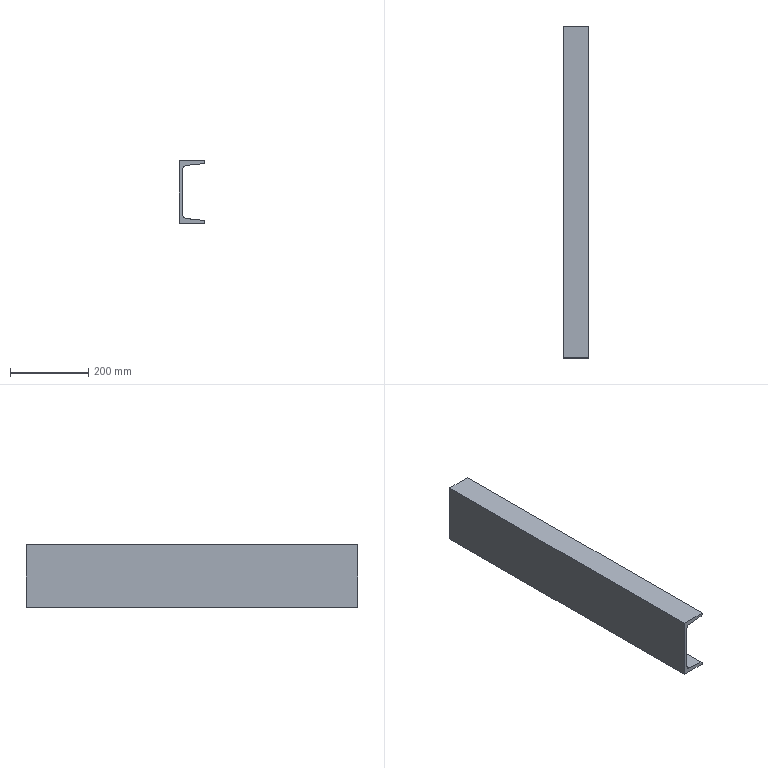Component | SolidWorks | NitrogenSupportChannelSteel65016a-2-331MachineTool-1 | 1 solid | 16 faces | box 65 x 850 x 160 mm | volume 2137912 mm3 | plane 10 | cylinder 6 | commonest cylinder face diameters 5 x2 20 x2 10 x2
build123d program:
from build123d import *

# Parameters (mm, degrees)
BOSS_EXTRUDE1_DEPTH    = 850
M6_TAPPED_HOLE1_REACH  = 866.871
M6_TAPPED_HOLE1_BORE_R = 2.5


with BuildPart() as part:
    # Sketch1 → Boss-Extrude1 (new body)
    with BuildSketch(Plane(origin=(0, 0, 0), x_dir=(-1, 0, 0), z_dir=(0, 0, -1))):
        with BuildLine():
            Line((-8.5, 138.125), (-8.5, 21.875))
            ThreePointArc((-8.5, 21.875), (-11.085, 15.165), (-17.505, 11.925))
            Line((-17.505, 11.925), (-60.498, 7.625))
            ThreePointArc((-60.498, 7.625), (-63.707, 6.005), (-65, 2.65))
            Line((-65, 2.65), (-65, 0))
            Line((-65, 0), (0, 0))
            Line((0, 0), (0, 160))
            Line((0, 160), (-65, 160))
            Line((-65, 160), (-65, 157.35))
            ThreePointArc((-65, 157.35), (-63.707, 153.995), (-60.498, 152.375))
            Line((-60.498, 152.375), (-17.505, 148.075))
            ThreePointArc((-17.505, 148.075), (-11.085, 144.835), (-8.5, 138.125))
        make_face()
    extrude(amount=-BOSS_EXTRUDE1_DEPTH)

    # M6 Tapped Hole1 bore → M6 Tapped Hole1 (cut, up to next)
    with BuildSketch(Plane(origin=(1.354, 13.54, 0), x_dir=(0.995, -0.0995, 0), z_dir=(0.0995, 0.995, 0)), mode=Mode.PRIVATE) as m6_tapped_hole1_sk1:
        with Locations((39.487, -548.988)):
            Circle(M6_TAPPED_HOLE1_BORE_R)
    m6_tapped_hole1_tool1 = extrude(m6_tapped_hole1_sk1.sketch, amount=-M6_TAPPED_HOLE1_REACH, mode=Mode.PRIVATE) & part.part
    add(m6_tapped_hole1_tool1.solids().sort_by_distance((40.645, 9.61, 548.988))[0], mode=Mode.SUBTRACT)


solid = part.part

# Placed as in the assembly
solid = solid.moved(Location((-286.681, 723.438, 590), (90, 0, 0)))
STEP:
#1=CARTESIAN_POINT('',(-9.823,6.868,23.228));
#2=VERTEX_POINT('',#1);
#3=CARTESIAN_POINT('',(-9.625,6.868,23.228));
#4=VERTEX_POINT('',#3);
#5=CARTESIAN_POINT('',(-9.823,6.868,23.228));
#6=CARTESIAN_POINT('',(-9.823,7.065,23.228));
#7=CARTESIAN_POINT('',(-9.625,7.065,23.228));
#8=CARTESIAN_POINT('',(-9.625,6.868,23.228));
#9=(BOUNDED_CURVE()B_SPLINE_CURVE(3,(#5,#6,#7,#8),.UNSPECIFIED.,.F.,.T.)B_SPLINE_CURVE_WITH_KNOTS((4,4),(3.142,6.283),.UNSPECIFIED.)CURVE()GEOMETRIC_REPRESENTATION_ITEM()RATIONAL_B_SPLINE_CURVE((1.,0.3333,0.3333,1.))REPRESENTATION_ITEM(''));
#10=EDGE_CURVE('',#2,#4,#9,.T.);
#11=ORIENTED_EDGE('',*,*,#10,.T.);
#12=CARTESIAN_POINT('',(-9.589,6.868,23.597));
#13=VERTEX_POINT('',#12);
#14=CARTESIAN_POINT('',(-9.589,6.868,23.597));
#15=DIRECTION('',(0.0995,-0.,0.995));
#16=VECTOR('',#15,39.37);
#17=LINE('',#14,#16);
#18=EDGE_CURVE('',#4,#13,#17,.T.);
#19=ORIENTED_EDGE('',*,*,#18,.T.);
#20=CARTESIAN_POINT('',(-9.784,6.868,23.617));
#21=VERTEX_POINT('',#20);
#22=CARTESIAN_POINT('',(-9.686,6.868,23.607));
#23=DIRECTION('',(0.0995,-0.,0.995));
#24=DIRECTION('',(-0.995,0.,0.0995));
#25=AXIS2_PLACEMENT_3D('',#22,#23,#24);
#26=CIRCLE('',#25,0.09843);
#27=EDGE_CURVE('',#13,#21,#26,.T.);
#28=ORIENTED_EDGE('',*,*,#27,.T.);
#29=CARTESIAN_POINT('',(-9.784,6.868,23.617));
#30=DIRECTION('',(0.0995,-0.,0.995));
#31=VECTOR('',#30,39.37);
#32=LINE('',#29,#31);
#33=EDGE_CURVE('',#2,#21,#32,.T.);
#34=ORIENTED_EDGE('',*,*,#33,.F.);
#35=EDGE_LOOP('',(#11,#19,#28,#34));
#36=FACE_OUTER_BOUND('',#35,.T.);
#37=CARTESIAN_POINT('',(-9.686,6.868,23.607));
#38=DIRECTION('',(0.0995,-0.,0.995));
#39=DIRECTION('',(-0.995,0.,0.0995));
#40=AXIS2_PLACEMENT_3D('',#37,#38,#39);
#41=CYLINDRICAL_SURFACE('',#40,0.09843);
#42=ADVANCED_FACE('',(#36),#41,.F.);
#43=CARTESIAN_POINT('',(-10.597,28.482,29.058));
#44=VERTEX_POINT('',#43);
#45=CARTESIAN_POINT('',(-10.952,28.482,28.666));
#46=VERTEX_POINT('',#45);
#47=CARTESIAN_POINT('',(-10.558,28.482,28.666));
#48=DIRECTION('',(-0.,-1.,-0.));
#49=DIRECTION('',(1.,0.,0.));
#50=AXIS2_PLACEMENT_3D('',#47,#48,#49);
#51=CIRCLE('',#50,0.3937);
#52=EDGE_CURVE('',#44,#46,#51,.T.);
#53=ORIENTED_EDGE('',*,*,#52,.F.);
#54=CARTESIAN_POINT('',(-10.597,-4.983,29.058));
#55=VERTEX_POINT('',#54);
#56=CARTESIAN_POINT('',(-10.597,-4.983,29.058));
#57=DIRECTION('',(0.,1.,0.));
#58=VECTOR('',#57,39.37);
#59=LINE('',#56,#58);
#60=EDGE_CURVE('',#55,#44,#59,.T.);
#61=ORIENTED_EDGE('',*,*,#60,.F.);
#62=CARTESIAN_POINT('',(-10.952,-4.983,28.666));
#63=VERTEX_POINT('',#62);
#64=CARTESIAN_POINT('',(-10.558,-4.983,28.666));
#65=DIRECTION('',(-0.,-1.,-0.));
#66=DIRECTION('',(1.,0.,0.));
#67=AXIS2_PLACEMENT_3D('',#64,#65,#66);
#68=CIRCLE('',#67,0.3937);
#69=EDGE_CURVE('',#55,#63,#68,.T.);
#70=ORIENTED_EDGE('',*,*,#69,.T.);
#71=CARTESIAN_POINT('',(-10.952,-4.983,28.666));
#72=DIRECTION('',(0.,1.,0.));
#73=VECTOR('',#72,39.37);
#74=LINE('',#71,#73);
#75=EDGE_CURVE('',#63,#46,#74,.T.);
#76=ORIENTED_EDGE('',*,*,#75,.T.);
#77=EDGE_LOOP('',(#53,#61,#70,#76));
#78=FACE_OUTER_BOUND('',#77,.T.);
#79=CARTESIAN_POINT('',(-10.558,-4.983,28.666));
#80=DIRECTION('',(0.,1.,0.));
#81=DIRECTION('',(-1.,0.,0.));
#82=AXIS2_PLACEMENT_3D('',#79,#80,#81);
#83=CYLINDRICAL_SURFACE('',#82,0.3937);
#84=ADVANCED_FACE('',(#78),#83,.F.);
#85=CARTESIAN_POINT('',(-8.905,28.482,29.227));
#86=VERTEX_POINT('',#85);
#87=CARTESIAN_POINT('',(-8.905,28.482,29.227));
#88=DIRECTION('',(-0.995,0.,-0.0995));
#89=VECTOR('',#88,39.37);
#90=LINE('',#87,#89);
#91=EDGE_CURVE('',#86,#44,#90,.T.);
#92=ORIENTED_EDGE('',*,*,#91,.F.);
#93=CARTESIAN_POINT('',(-8.905,-4.983,29.227));
#94=VERTEX_POINT('',#93);
#95=CARTESIAN_POINT('',(-8.905,-4.983,29.227));
#96=DIRECTION('',(0.,1.,0.));
#97=VECTOR('',#96,39.37);
#98=LINE('',#95,#97);
#99=EDGE_CURVE('',#94,#86,#98,.T.);
#100=ORIENTED_EDGE('',*,*,#99,.F.);
#101=CARTESIAN_POINT('',(-8.905,-4.983,29.227));
#102=DIRECTION('',(-0.995,0.,-0.0995));
#103=VECTOR('',#102,39.37);
#104=LINE('',#101,#103);
#105=EDGE_CURVE('',#94,#55,#104,.T.);
#106=ORIENTED_EDGE('',*,*,#105,.T.);
#107=ORIENTED_EDGE('',*,*,#60,.T.);
#108=EDGE_LOOP('',(#92,#100,#106,#107));
#109=FACE_OUTER_BOUND('',#108,.T.);
#110=CARTESIAN_POINT('',(-8.905,-4.983,29.227));
#111=DIRECTION('',(0.0995,0.,-0.995));
#112=DIRECTION('',(0.995,-0.,0.0995));
#113=AXIS2_PLACEMENT_3D('',#110,#111,#112);
#114=PLANE('',#113);
#115=ADVANCED_FACE('',(#109),#114,.T.);
#116=CARTESIAN_POINT('',(-8.728,28.482,29.423));
#117=VERTEX_POINT('',#116);
#118=CARTESIAN_POINT('',(-8.924,28.482,29.423));
#119=DIRECTION('',(0.,1.,0.));
#120=DIRECTION('',(-1.,0.,0.));
#121=AXIS2_PLACEMENT_3D('',#118,#119,#120);
#122=CIRCLE('',#121,0.1969);
#123=EDGE_CURVE('',#117,#86,#122,.T.);
#124=ORIENTED_EDGE('',*,*,#123,.F.);
#125=CARTESIAN_POINT('',(-8.728,-4.983,29.423));
#126=VERTEX_POINT('',#125);
#127=CARTESIAN_POINT('',(-8.728,-4.983,29.423));
#128=DIRECTION('',(0.,1.,0.));
#129=VECTOR('',#128,39.37);
#130=LINE('',#127,#129);
#131=EDGE_CURVE('',#126,#117,#130,.T.);
#132=ORIENTED_EDGE('',*,*,#131,.F.);
#133=CARTESIAN_POINT('',(-8.924,-4.983,29.423));
#134=DIRECTION('',(0.,1.,0.));
#135=DIRECTION('',(-1.,0.,0.));
#136=AXIS2_PLACEMENT_3D('',#133,#134,#135);
#137=CIRCLE('',#136,0.1969);
#138=EDGE_CURVE('',#126,#94,#137,.T.);
#139=ORIENTED_EDGE('',*,*,#138,.T.);
#140=ORIENTED_EDGE('',*,*,#99,.T.);
#141=EDGE_LOOP('',(#124,#132,#139,#140));
#142=FACE_OUTER_BOUND('',#141,.T.);
#143=CARTESIAN_POINT('',(-8.924,-4.983,29.423));
#144=DIRECTION('',(0.,1.,0.));
#145=DIRECTION('',(-1.,0.,0.));
#146=AXIS2_PLACEMENT_3D('',#143,#144,#145);
#147=CYLINDRICAL_SURFACE('',#146,0.1969);
#148=ADVANCED_FACE('',(#142),#147,.T.);
#149=CARTESIAN_POINT('',(-8.728,28.482,29.528));
#150=VERTEX_POINT('',#149);
#151=CARTESIAN_POINT('',(-8.728,28.482,29.528));
#152=DIRECTION('',(0.,0.,-1.));
#153=VECTOR('',#152,39.37);
#154=LINE('',#151,#153);
#155=EDGE_CURVE('',#150,#117,#154,.T.);
#156=ORIENTED_EDGE('',*,*,#155,.F.);
#157=CARTESIAN_POINT('',(-8.728,-4.983,29.528));
#158=VERTEX_POINT('',#157);
#159=CARTESIAN_POINT('',(-8.728,-4.983,29.528));
#160=DIRECTION('',(0.,1.,0.));
#161=VECTOR('',#160,39.37);
#162=LINE('',#159,#161);
#163=EDGE_CURVE('',#158,#150,#162,.T.);
#164=ORIENTED_EDGE('',*,*,#163,.F.);
#165=CARTESIAN_POINT('',(-8.728,-4.983,29.528));
#166=DIRECTION('',(0.,0.,-1.));
#167=VECTOR('',#166,39.37);
#168=LINE('',#165,#167);
#169=EDGE_CURVE('',#158,#126,#168,.T.);
#170=ORIENTED_EDGE('',*,*,#169,.T.);
#171=ORIENTED_EDGE('',*,*,#131,.T.);
#172=EDGE_LOOP('',(#156,#164,#170,#171));
#173=FACE_OUTER_BOUND('',#172,.T.);
#174=CARTESIAN_POINT('',(-8.728,-4.983,29.528));
#175=DIRECTION('',(1.,-0.,0.));
#176=DIRECTION('',(0.,1.,0.));
#177=AXIS2_PLACEMENT_3D('',#174,#175,#176);
#178=PLANE('',#177);
#179=ADVANCED_FACE('',(#173),#178,.T.);
#180=CARTESIAN_POINT('',(-11.287,28.482,29.528));
#181=VERTEX_POINT('',#180);
#182=CARTESIAN_POINT('',(-11.287,28.482,29.528));
#183=DIRECTION('',(1.,0.,0.));
#184=VECTOR('',#183,39.37);
#185=LINE('',#182,#184);
#186=EDGE_CURVE('',#181,#150,#185,.T.);
#187=ORIENTED_EDGE('',*,*,#186,.F.);
#188=CARTESIAN_POINT('',(-11.287,-4.983,29.528));
#189=VERTEX_POINT('',#188);
#190=CARTESIAN_POINT('',(-11.287,-4.983,29.528));
#191=DIRECTION('',(0.,1.,0.));
#192=VECTOR('',#191,39.37);
#193=LINE('',#190,#192);
#194=EDGE_CURVE('',#189,#181,#193,.T.);
#195=ORIENTED_EDGE('',*,*,#194,.F.);
#196=CARTESIAN_POINT('',(-11.287,-4.983,29.528));
#197=DIRECTION('',(1.,0.,0.));
#198=VECTOR('',#197,39.37);
#199=LINE('',#196,#198);
#200=EDGE_CURVE('',#189,#158,#199,.T.);
#201=ORIENTED_EDGE('',*,*,#200,.T.);
#202=ORIENTED_EDGE('',*,*,#163,.T.);
#203=EDGE_LOOP('',(#187,#195,#201,#202));
#204=FACE_OUTER_BOUND('',#203,.T.);
#205=CARTESIAN_POINT('',(-11.287,-4.983,29.528));
#206=DIRECTION('',(-0.,-0.,1.));
#207=DIRECTION('',(-0.,-1.,-0.));
#208=AXIS2_PLACEMENT_3D('',#205,#206,#207);
#209=PLANE('',#208);
#210=ADVANCED_FACE('',(#204),#209,.T.);
#211=CARTESIAN_POINT('',(-11.287,28.482,23.228));
#212=VERTEX_POINT('',#211);
#213=CARTESIAN_POINT('',(-11.287,28.482,23.228));
#214=DIRECTION('',(-0.,-0.,1.));
#215=VECTOR('',#214,39.37);
#216=LINE('',#213,#215);
#217=EDGE_CURVE('',#212,#181,#216,.T.);
#218=ORIENTED_EDGE('',*,*,#217,.F.);
#219=CARTESIAN_POINT('',(-11.287,-4.983,23.228));
#220=VERTEX_POINT('',#219);
#221=CARTESIAN_POINT('',(-11.287,-4.983,23.228));
#222=DIRECTION('',(0.,1.,0.));
#223=VECTOR('',#222,39.37);
#224=LINE('',#221,#223);
#225=EDGE_CURVE('',#220,#212,#224,.T.);
#226=ORIENTED_EDGE('',*,*,#225,.F.);
#227=CARTESIAN_POINT('',(-11.287,-4.983,23.228));
#228=DIRECTION('',(-0.,-0.,1.));
#229=VECTOR('',#228,39.37);
#230=LINE('',#227,#229);
#231=EDGE_CURVE('',#220,#189,#230,.T.);
#232=ORIENTED_EDGE('',*,*,#231,.T.);
#233=ORIENTED_EDGE('',*,*,#194,.T.);
#234=EDGE_LOOP('',(#218,#226,#232,#233));
#235=FACE_OUTER_BOUND('',#234,.T.);
#236=CARTESIAN_POINT('',(-11.287,-4.983,23.228));
#237=DIRECTION('',(-1.,0.,-0.));
#238=DIRECTION('',(-0.,-1.,-0.));
#239=AXIS2_PLACEMENT_3D('',#236,#237,#238);
#240=PLANE('',#239);
#241=ADVANCED_FACE('',(#235),#240,.T.);
#242=ORIENTED_EDGE('',*,*,#10,.F.);
#243=CARTESIAN_POINT('',(-9.625,6.868,23.228));
#244=CARTESIAN_POINT('',(-9.625,6.671,23.228));
#245=CARTESIAN_POINT('',(-9.823,6.671,23.228));
#246=CARTESIAN_POINT('',(-9.823,6.868,23.228));
#247=(BOUNDED_CURVE()B_SPLINE_CURVE(3,(#243,#244,#245,#246),.UNSPECIFIED.,.F.,.T.)B_SPLINE_CURVE_WITH_KNOTS((4,4),(0.,3.142),.UNSPECIFIED.)CURVE()GEOMETRIC_REPRESENTATION_ITEM()RATIONAL_B_SPLINE_CURVE((1.,0.3333,0.3333,1.))REPRESENTATION_ITEM(''));
#248=EDGE_CURVE('',#4,#2,#247,.T.);
#249=ORIENTED_EDGE('',*,*,#248,.F.);
#250=EDGE_LOOP('',(#242,#249));
#251=FACE_BOUND('',#250,.T.);
#252=CARTESIAN_POINT('',(-8.728,28.482,23.228));
#253=VERTEX_POINT('',#252);
#254=CARTESIAN_POINT('',(-8.728,28.482,23.228));
#255=DIRECTION('',(-1.,-0.,-0.));
#256=VECTOR('',#255,39.37);
#257=LINE('',#254,#256);
#258=EDGE_CURVE('',#253,#212,#257,.T.);
#259=ORIENTED_EDGE('',*,*,#258,.F.);
#260=CARTESIAN_POINT('',(-8.728,-4.983,23.228));
#261=VERTEX_POINT('',#260);
#262=CARTESIAN_POINT('',(-8.728,-4.983,23.228));
#263=DIRECTION('',(0.,1.,0.));
#264=VECTOR('',#263,39.37);
#265=LINE('',#262,#264);
#266=EDGE_CURVE('',#261,#253,#265,.T.);
#267=ORIENTED_EDGE('',*,*,#266,.F.);
#268=CARTESIAN_POINT('',(-8.728,-4.983,23.228));
#269=DIRECTION('',(-1.,-0.,-0.));
#270=VECTOR('',#269,39.37);
#271=LINE('',#268,#270);
#272=EDGE_CURVE('',#261,#220,#271,.T.);
#273=ORIENTED_EDGE('',*,*,#272,.T.);
#274=ORIENTED_EDGE('',*,*,#225,.T.);
#275=EDGE_LOOP('',(#259,#267,#273,#274));
#276=FACE_OUTER_BOUND('',#275,.T.);
#277=CARTESIAN_POINT('',(-8.728,-4.983,23.228));
#278=DIRECTION('',(0.,0.,-1.));
#279=DIRECTION('',(0.,1.,0.));
#280=AXIS2_PLACEMENT_3D('',#277,#278,#279);
#281=PLANE('',#280);
#282=ADVANCED_FACE('',(#251,#276),#281,.T.);
#283=CARTESIAN_POINT('',(-8.728,28.482,23.333));
#284=VERTEX_POINT('',#283);
#285=CARTESIAN_POINT('',(-8.728,28.482,23.333));
#286=DIRECTION('',(0.,0.,-1.));
#287=VECTOR('',#286,39.37);
#288=LINE('',#285,#287);
#289=EDGE_CURVE('',#284,#253,#288,.T.);
#290=ORIENTED_EDGE('',*,*,#289,.F.);
#291=CARTESIAN_POINT('',(-8.728,-4.983,23.333));
#292=VERTEX_POINT('',#291);
#293=CARTESIAN_POINT('',(-8.728,-4.983,23.333));
#294=DIRECTION('',(0.,1.,0.));
#295=VECTOR('',#294,39.37);
#296=LINE('',#293,#295);
#297=EDGE_CURVE('',#292,#284,#296,.T.);
#298=ORIENTED_EDGE('',*,*,#297,.F.);
#299=CARTESIAN_POINT('',(-8.728,-4.983,23.333));
#300=DIRECTION('',(0.,0.,-1.));
#301=VECTOR('',#300,39.37);
#302=LINE('',#299,#301);
#303=EDGE_CURVE('',#292,#261,#302,.T.);
#304=ORIENTED_EDGE('',*,*,#303,.T.);
#305=ORIENTED_EDGE('',*,*,#266,.T.);
#306=EDGE_LOOP('',(#290,#298,#304,#305));
#307=FACE_OUTER_BOUND('',#306,.T.);
#308=CARTESIAN_POINT('',(-8.728,-4.983,23.333));
#309=DIRECTION('',(1.,-0.,0.));
#310=DIRECTION('',(0.,1.,0.));
#311=AXIS2_PLACEMENT_3D('',#308,#309,#310);
#312=PLANE('',#311);
#313=ADVANCED_FACE('',(#307),#312,.T.);
#314=CARTESIAN_POINT('',(-8.905,28.482,23.529));
#315=VERTEX_POINT('',#314);
#316=CARTESIAN_POINT('',(-8.924,28.482,23.333));
#317=DIRECTION('',(0.,1.,0.));
#318=DIRECTION('',(-1.,0.,0.));
#319=AXIS2_PLACEMENT_3D('',#316,#317,#318);
#320=CIRCLE('',#319,0.1969);
#321=EDGE_CURVE('',#315,#284,#320,.T.);
#322=ORIENTED_EDGE('',*,*,#321,.F.);
#323=CARTESIAN_POINT('',(-8.905,-4.983,23.529));
#324=VERTEX_POINT('',#323);
#325=CARTESIAN_POINT('',(-8.905,-4.983,23.529));
#326=DIRECTION('',(0.,1.,0.));
#327=VECTOR('',#326,39.37);
#328=LINE('',#325,#327);
#329=EDGE_CURVE('',#324,#315,#328,.T.);
#330=ORIENTED_EDGE('',*,*,#329,.F.);
#331=CARTESIAN_POINT('',(-8.924,-4.983,23.333));
#332=DIRECTION('',(0.,1.,0.));
#333=DIRECTION('',(-1.,0.,0.));
#334=AXIS2_PLACEMENT_3D('',#331,#332,#333);
#335=CIRCLE('',#334,0.1969);
#336=EDGE_CURVE('',#324,#292,#335,.T.);
#337=ORIENTED_EDGE('',*,*,#336,.T.);
#338=ORIENTED_EDGE('',*,*,#297,.T.);
#339=EDGE_LOOP('',(#322,#330,#337,#338));
#340=FACE_OUTER_BOUND('',#339,.T.);
#341=CARTESIAN_POINT('',(-8.924,-4.983,23.333));
#342=DIRECTION('',(0.,1.,0.));
#343=DIRECTION('',(-1.,0.,0.));
#344=AXIS2_PLACEMENT_3D('',#341,#342,#343);
#345=CYLINDRICAL_SURFACE('',#344,0.1969);
#346=ADVANCED_FACE('',(#340),#345,.T.);
#347=CARTESIAN_POINT('',(-9.686,6.868,23.607));
#348=DIRECTION('',(0.0995,-0.,0.995));
#349=DIRECTION('',(-0.995,0.,0.0995));
#350=AXIS2_PLACEMENT_3D('',#347,#348,#349);
#351=CIRCLE('',#350,0.09843);
#352=EDGE_CURVE('',#21,#13,#351,.T.);
#353=ORIENTED_EDGE('',*,*,#352,.F.);
#354=ORIENTED_EDGE('',*,*,#27,.F.);
#355=EDGE_LOOP('',(#353,#354));
#356=FACE_BOUND('',#355,.T.);
#357=CARTESIAN_POINT('',(-10.597,28.482,23.698));
#358=VERTEX_POINT('',#357);
#359=CARTESIAN_POINT('',(-10.597,28.482,23.698));
#360=DIRECTION('',(0.995,0.,-0.0995));
#361=VECTOR('',#360,39.37);
#362=LINE('',#359,#361);
#363=EDGE_CURVE('',#358,#315,#362,.T.);
#364=ORIENTED_EDGE('',*,*,#363,.F.);
#365=CARTESIAN_POINT('',(-10.597,-4.983,23.698));
#366=VERTEX_POINT('',#365);
#367=CARTESIAN_POINT('',(-10.597,-4.983,23.698));
#368=DIRECTION('',(0.,1.,0.));
#369=VECTOR('',#368,39.37);
#370=LINE('',#367,#369);
#371=EDGE_CURVE('',#366,#358,#370,.T.);
#372=ORIENTED_EDGE('',*,*,#371,.F.);
#373=CARTESIAN_POINT('',(-10.597,-4.983,23.698));
#374=DIRECTION('',(0.995,0.,-0.0995));
#375=VECTOR('',#374,39.37);
#376=LINE('',#373,#375);
#377=EDGE_CURVE('',#366,#324,#376,.T.);
#378=ORIENTED_EDGE('',*,*,#377,.T.);
#379=ORIENTED_EDGE('',*,*,#329,.T.);
#380=EDGE_LOOP('',(#364,#372,#378,#379));
#381=FACE_OUTER_BOUND('',#380,.T.);
#382=CARTESIAN_POINT('',(-10.597,-4.983,23.698));
#383=DIRECTION('',(0.0995,-0.,0.995));
#384=DIRECTION('',(-0.995,-0.,0.0995));
#385=AXIS2_PLACEMENT_3D('',#382,#383,#384);
#386=PLANE('',#385);
#387=ADVANCED_FACE('',(#356,#381),#386,.T.);
#388=CARTESIAN_POINT('',(-10.952,28.482,24.09));
#389=VERTEX_POINT('',#388);
#390=CARTESIAN_POINT('',(-10.558,28.482,24.09));
#391=DIRECTION('',(-0.,-1.,-0.));
#392=DIRECTION('',(1.,0.,0.));
#393=AXIS2_PLACEMENT_3D('',#390,#391,#392);
#394=CIRCLE('',#393,0.3937);
#395=EDGE_CURVE('',#389,#358,#394,.T.);
#396=ORIENTED_EDGE('',*,*,#395,.F.);
#397=CARTESIAN_POINT('',(-10.952,-4.983,24.09));
#398=VERTEX_POINT('',#397);
#399=CARTESIAN_POINT('',(-10.952,-4.983,24.09));
#400=DIRECTION('',(0.,1.,0.));
#401=VECTOR('',#400,39.37);
#402=LINE('',#399,#401);
#403=EDGE_CURVE('',#398,#389,#402,.T.);
#404=ORIENTED_EDGE('',*,*,#403,.F.);
#405=CARTESIAN_POINT('',(-10.558,-4.983,24.09));
#406=DIRECTION('',(-0.,-1.,-0.));
#407=DIRECTION('',(1.,0.,0.));
#408=AXIS2_PLACEMENT_3D('',#405,#406,#407);
#409=CIRCLE('',#408,0.3937);
#410=EDGE_CURVE('',#398,#366,#409,.T.);
#411=ORIENTED_EDGE('',*,*,#410,.T.);
#412=ORIENTED_EDGE('',*,*,#371,.T.);
#413=EDGE_LOOP('',(#396,#404,#411,#412));
#414=FACE_OUTER_BOUND('',#413,.T.);
#415=CARTESIAN_POINT('',(-10.558,-4.983,24.09));
#416=DIRECTION('',(0.,1.,0.));
#417=DIRECTION('',(-1.,0.,0.));
#418=AXIS2_PLACEMENT_3D('',#415,#416,#417);
#419=CYLINDRICAL_SURFACE('',#418,0.3937);
#420=ADVANCED_FACE('',(#414),#419,.F.);
#421=CARTESIAN_POINT('',(-10.952,28.482,28.666));
#422=DIRECTION('',(0.,0.,-1.));
#423=VECTOR('',#422,39.37);
#424=LINE('',#421,#423);
#425=EDGE_CURVE('',#46,#389,#424,.T.);
#426=ORIENTED_EDGE('',*,*,#425,.F.);
#427=ORIENTED_EDGE('',*,*,#75,.F.);
#428=CARTESIAN_POINT('',(-10.952,-4.983,28.666));
#429=DIRECTION('',(0.,0.,-1.));
#430=VECTOR('',#429,39.37);
#431=LINE('',#428,#430);
#432=EDGE_CURVE('',#63,#398,#431,.T.);
#433=ORIENTED_EDGE('',*,*,#432,.T.);
#434=ORIENTED_EDGE('',*,*,#403,.T.);
#435=EDGE_LOOP('',(#426,#427,#433,#434));
#436=FACE_OUTER_BOUND('',#435,.T.);
#437=CARTESIAN_POINT('',(-10.952,-4.983,28.666));
#438=DIRECTION('',(1.,0.,0.));
#439=DIRECTION('',(-0.,-0.,1.));
#440=AXIS2_PLACEMENT_3D('',#437,#438,#439);
#441=PLANE('',#440);
#442=ADVANCED_FACE('',(#436),#441,.T.);
#443=ORIENTED_EDGE('',*,*,#69,.F.);
#444=ORIENTED_EDGE('',*,*,#105,.F.);
#445=ORIENTED_EDGE('',*,*,#138,.F.);
#446=ORIENTED_EDGE('',*,*,#169,.F.);
#447=ORIENTED_EDGE('',*,*,#200,.F.);
#448=ORIENTED_EDGE('',*,*,#231,.F.);
#449=ORIENTED_EDGE('',*,*,#272,.F.);
#450=ORIENTED_EDGE('',*,*,#303,.F.);
#451=ORIENTED_EDGE('',*,*,#336,.F.);
#452=ORIENTED_EDGE('',*,*,#377,.F.);
#453=ORIENTED_EDGE('',*,*,#410,.F.);
#454=ORIENTED_EDGE('',*,*,#432,.F.);
#455=EDGE_LOOP('',(#443,#444,#445,#446,#447,#448,#449,#450,#451,#452,#453,#454));
#456=FACE_OUTER_BOUND('',#455,.T.);
#457=CARTESIAN_POINT('',(-10.558,-4.983,28.666));
#458=DIRECTION('',(0.,-1.,-0.));
#459=DIRECTION('',(1.,0.,0.));
#460=AXIS2_PLACEMENT_3D('',#457,#458,#459);
#461=PLANE('',#460);
#462=ADVANCED_FACE('',(#456),#461,.T.);
#463=ORIENTED_EDGE('',*,*,#52,.T.);
#464=ORIENTED_EDGE('',*,*,#425,.T.);
#465=ORIENTED_EDGE('',*,*,#395,.T.);
#466=ORIENTED_EDGE('',*,*,#363,.T.);
#467=ORIENTED_EDGE('',*,*,#321,.T.);
#468=ORIENTED_EDGE('',*,*,#289,.T.);
#469=ORIENTED_EDGE('',*,*,#258,.T.);
#470=ORIENTED_EDGE('',*,*,#217,.T.);
#471=ORIENTED_EDGE('',*,*,#186,.T.);
#472=ORIENTED_EDGE('',*,*,#155,.T.);
#473=ORIENTED_EDGE('',*,*,#123,.T.);
#474=ORIENTED_EDGE('',*,*,#91,.T.);
#475=EDGE_LOOP('',(#463,#464,#465,#466,#467,#468,#469,#470,#471,#472,#473,#474));
#476=FACE_OUTER_BOUND('',#475,.T.);
#477=CARTESIAN_POINT('',(-10.558,28.482,28.666));
#478=DIRECTION('',(0.,-1.,-0.));
#479=DIRECTION('',(1.,0.,0.));
#480=AXIS2_PLACEMENT_3D('',#477,#478,#479);
#481=PLANE('',#480);
#482=ADVANCED_FACE('',(#476),#481,.F.);
#483=ORIENTED_EDGE('',*,*,#18,.F.);
#484=ORIENTED_EDGE('',*,*,#248,.T.);
#485=ORIENTED_EDGE('',*,*,#33,.T.);
#486=ORIENTED_EDGE('',*,*,#352,.T.);
#487=EDGE_LOOP('',(#483,#484,#485,#486));
#488=FACE_OUTER_BOUND('',#487,.T.);
#489=CARTESIAN_POINT('',(-9.686,6.868,23.607));
#490=DIRECTION('',(0.0995,-0.,0.995));
#491=DIRECTION('',(-0.995,0.,0.0995));
#492=AXIS2_PLACEMENT_3D('',#489,#490,#491);
#493=CYLINDRICAL_SURFACE('',#492,0.09843);
#494=ADVANCED_FACE('',(#488),#493,.F.);
#495=CLOSED_SHELL('',(#42,#84,#115,#148,#179,#210,#241,#282,#313,#346,#387,#420,#442,#462,#482,#494));
#496=MANIFOLD_SOLID_BREP('',#495);
#497=CARTESIAN_POINT('',(0.,0.,0.));
#498=DIRECTION('',(0.,0.,1.));
#499=DIRECTION('',(1.,0.,0.));
#500=AXIS2_PLACEMENT_3D('',#497,#498,#499);
#501=(LENGTH_UNIT()NAMED_UNIT(*)SI_UNIT($,.METRE.));
#502=LENGTH_MEASURE_WITH_UNIT(LENGTH_MEASURE(0.0254),#501);
#503=DIMENSIONAL_EXPONENTS(1.,0.,0.,0.,0.,0.,0.);
#504=(CONVERSION_BASED_UNIT('',#502)LENGTH_UNIT()NAMED_UNIT(#503));
#505=UNCERTAINTY_MEASURE_WITH_UNIT(LENGTH_MEASURE(0.00001),#504,'','');
#506=(NAMED_UNIT(*)PLANE_ANGLE_UNIT()SI_UNIT($,.RADIAN.));
#507=(NAMED_UNIT(*)SI_UNIT($,.STERADIAN.)SOLID_ANGLE_UNIT());
#508=(GEOMETRIC_REPRESENTATION_CONTEXT(3)GLOBAL_UNCERTAINTY_ASSIGNED_CONTEXT((#505))GLOBAL_UNIT_ASSIGNED_CONTEXT((#504,#506,#507))REPRESENTATION_CONTEXT('',''));
#509=ADVANCED_BREP_SHAPE_REPRESENTATION('',(#496,#500),#508);
#510=COLOUR_RGB('',0.7922,0.8196,0.9333);
#511=FILL_AREA_STYLE_COLOUR('',#510);
#512=FILL_AREA_STYLE('',(#511));
#513=SURFACE_STYLE_FILL_AREA(#512);
#514=SURFACE_SIDE_STYLE('',(#513));
#515=SURFACE_STYLE_USAGE(.BOTH.,#514);
#516=PRESENTATION_STYLE_ASSIGNMENT((#515));
#517=STYLED_ITEM('',(#516),#496);
#518=(LENGTH_UNIT()NAMED_UNIT(*)SI_UNIT($,.METRE.));
#519=LENGTH_MEASURE_WITH_UNIT(LENGTH_MEASURE(0.0254),#518);
#520=DIMENSIONAL_EXPONENTS(1.,0.,0.,0.,0.,0.,0.);
#521=(CONVERSION_BASED_UNIT('',#519)LENGTH_UNIT()NAMED_UNIT(#520));
#522=UNCERTAINTY_MEASURE_WITH_UNIT(LENGTH_MEASURE(0.00001),#521,'','');
#523=(NAMED_UNIT(*)PLANE_ANGLE_UNIT()SI_UNIT($,.RADIAN.));
#524=(NAMED_UNIT(*)SI_UNIT($,.STERADIAN.)SOLID_ANGLE_UNIT());
#525=(GEOMETRIC_REPRESENTATION_CONTEXT(3)GLOBAL_UNCERTAINTY_ASSIGNED_CONTEXT((#522))GLOBAL_UNIT_ASSIGNED_CONTEXT((#521,#523,#524))REPRESENTATION_CONTEXT('',''));
#526=MECHANICAL_DESIGN_GEOMETRIC_PRESENTATION_REPRESENTATION('',(#517),#525);
#527=PRESENTATION_LAYER_ASSIGNMENT('','',(#517));